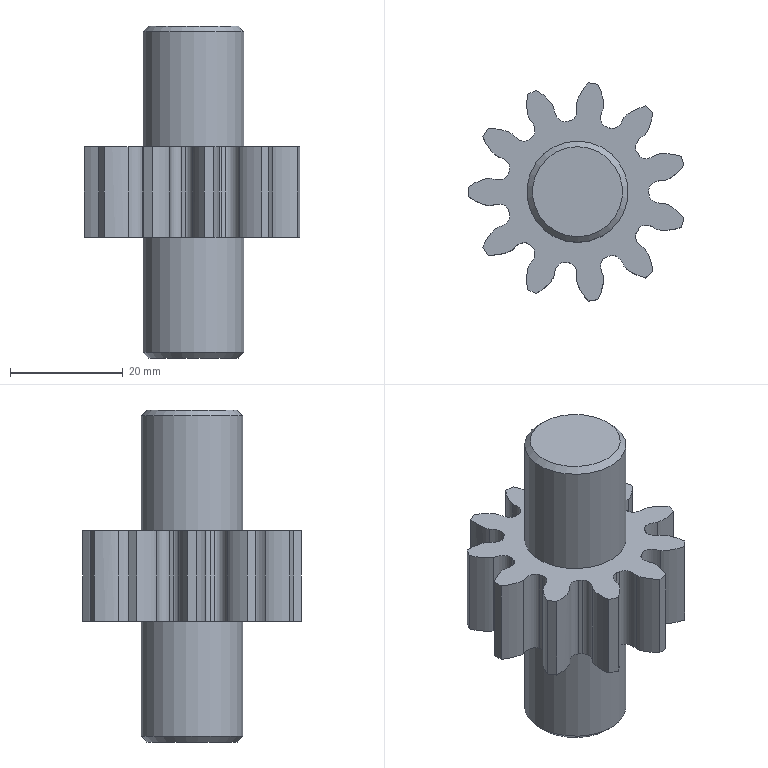Component | NX | 4 | 1 solid | 74 faces | volume 23890 mm3 | spline 55 | cylinder 13 | plane 4 | cone 2 | commonest cylinder face diameters 25.4 x11 18 x2